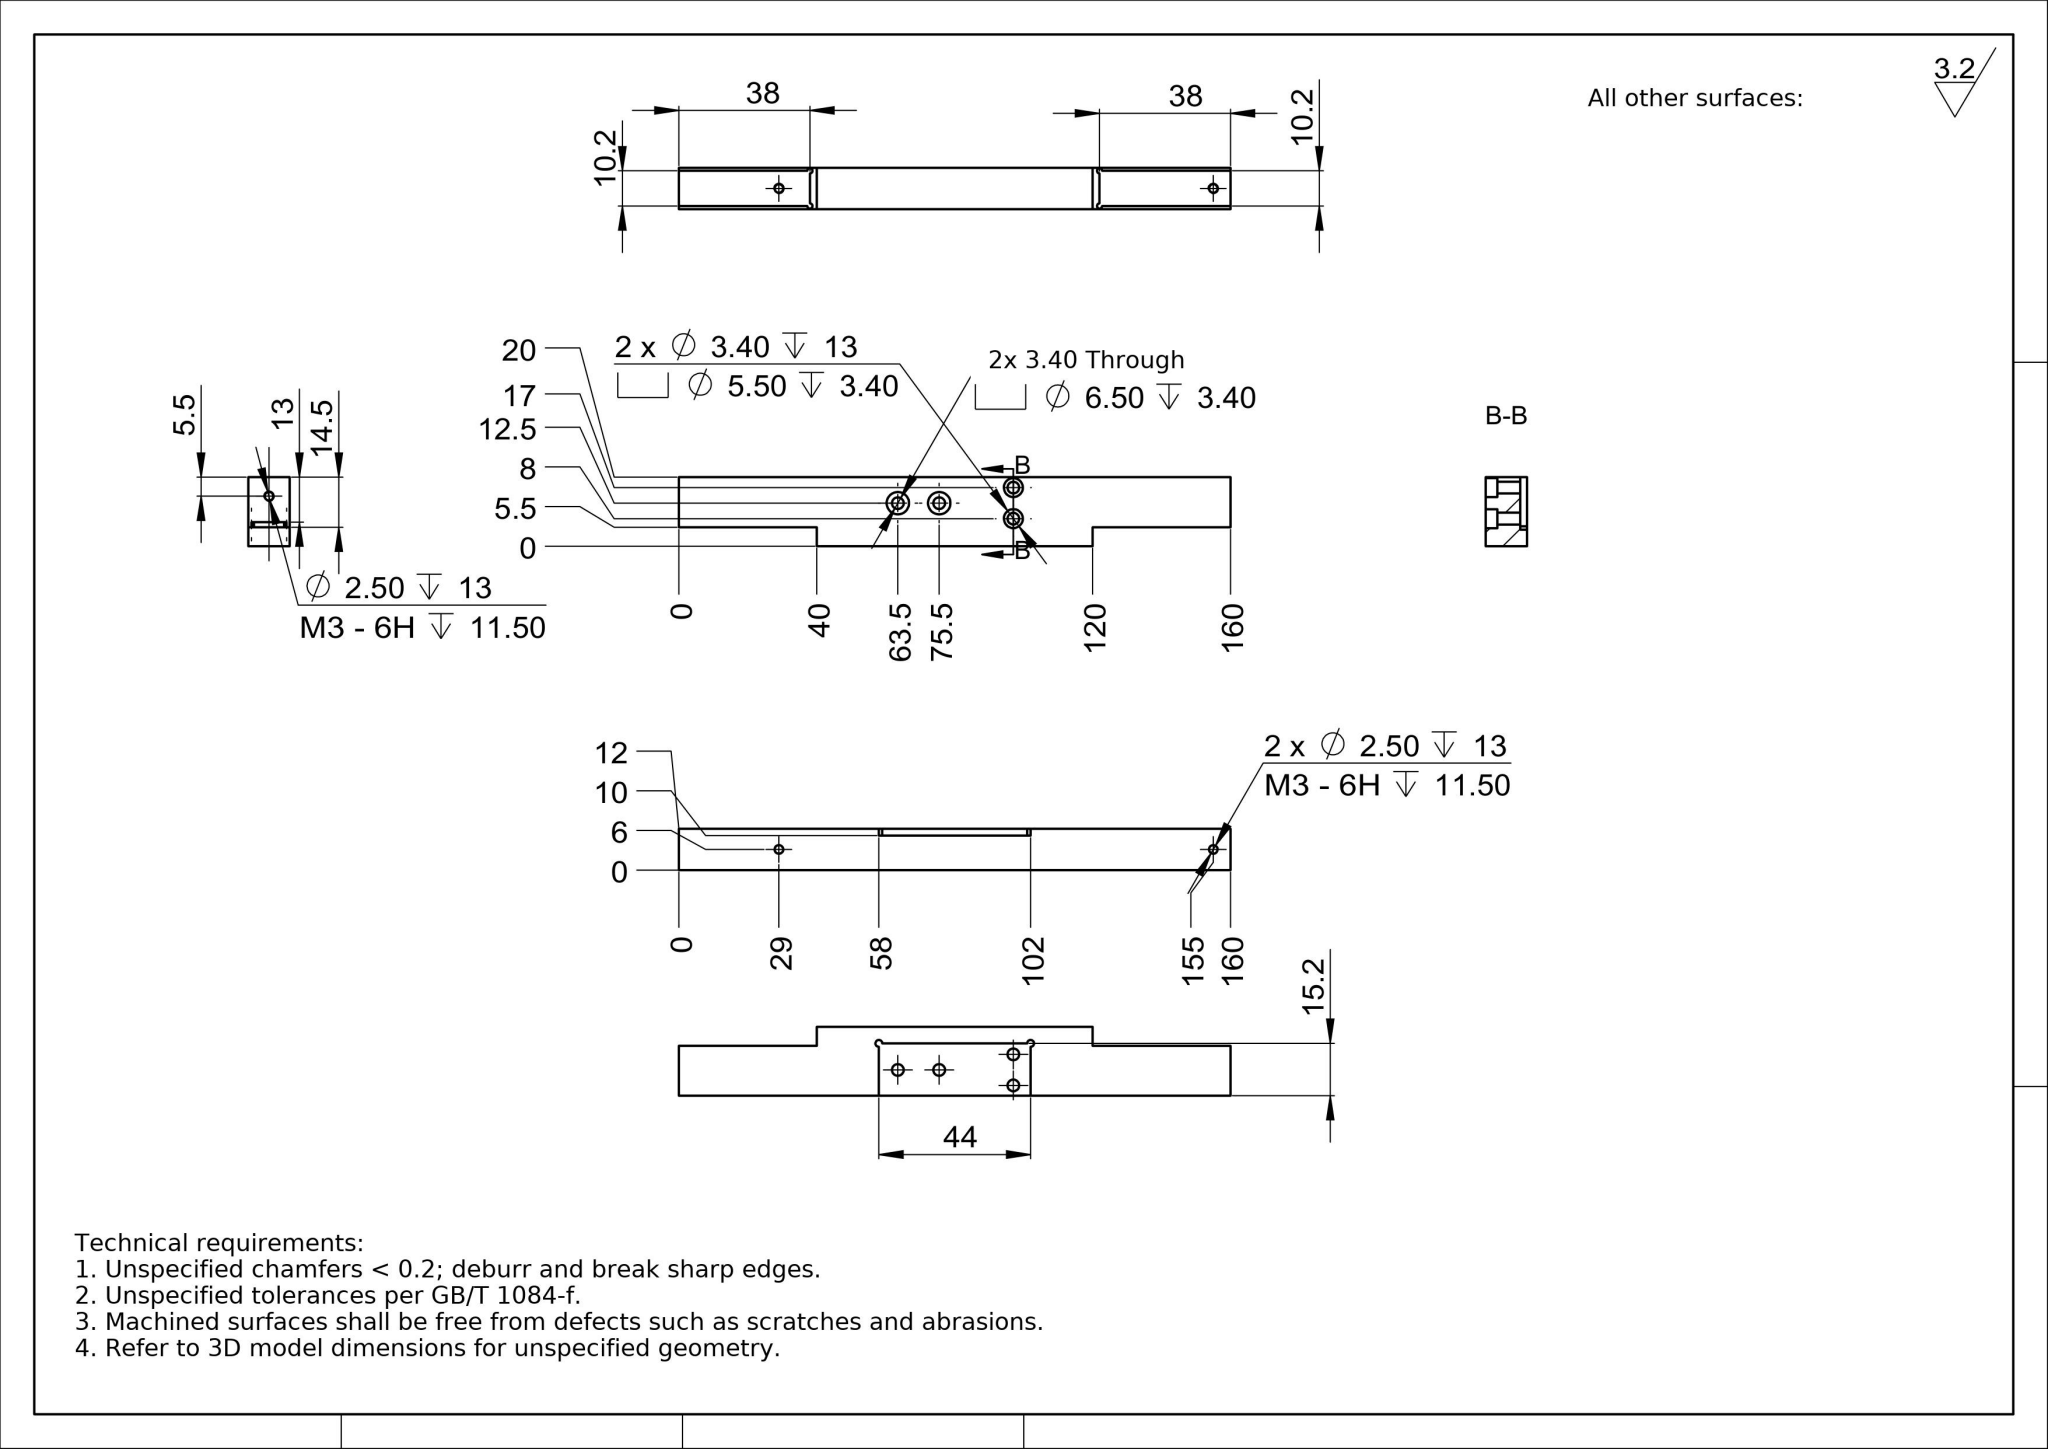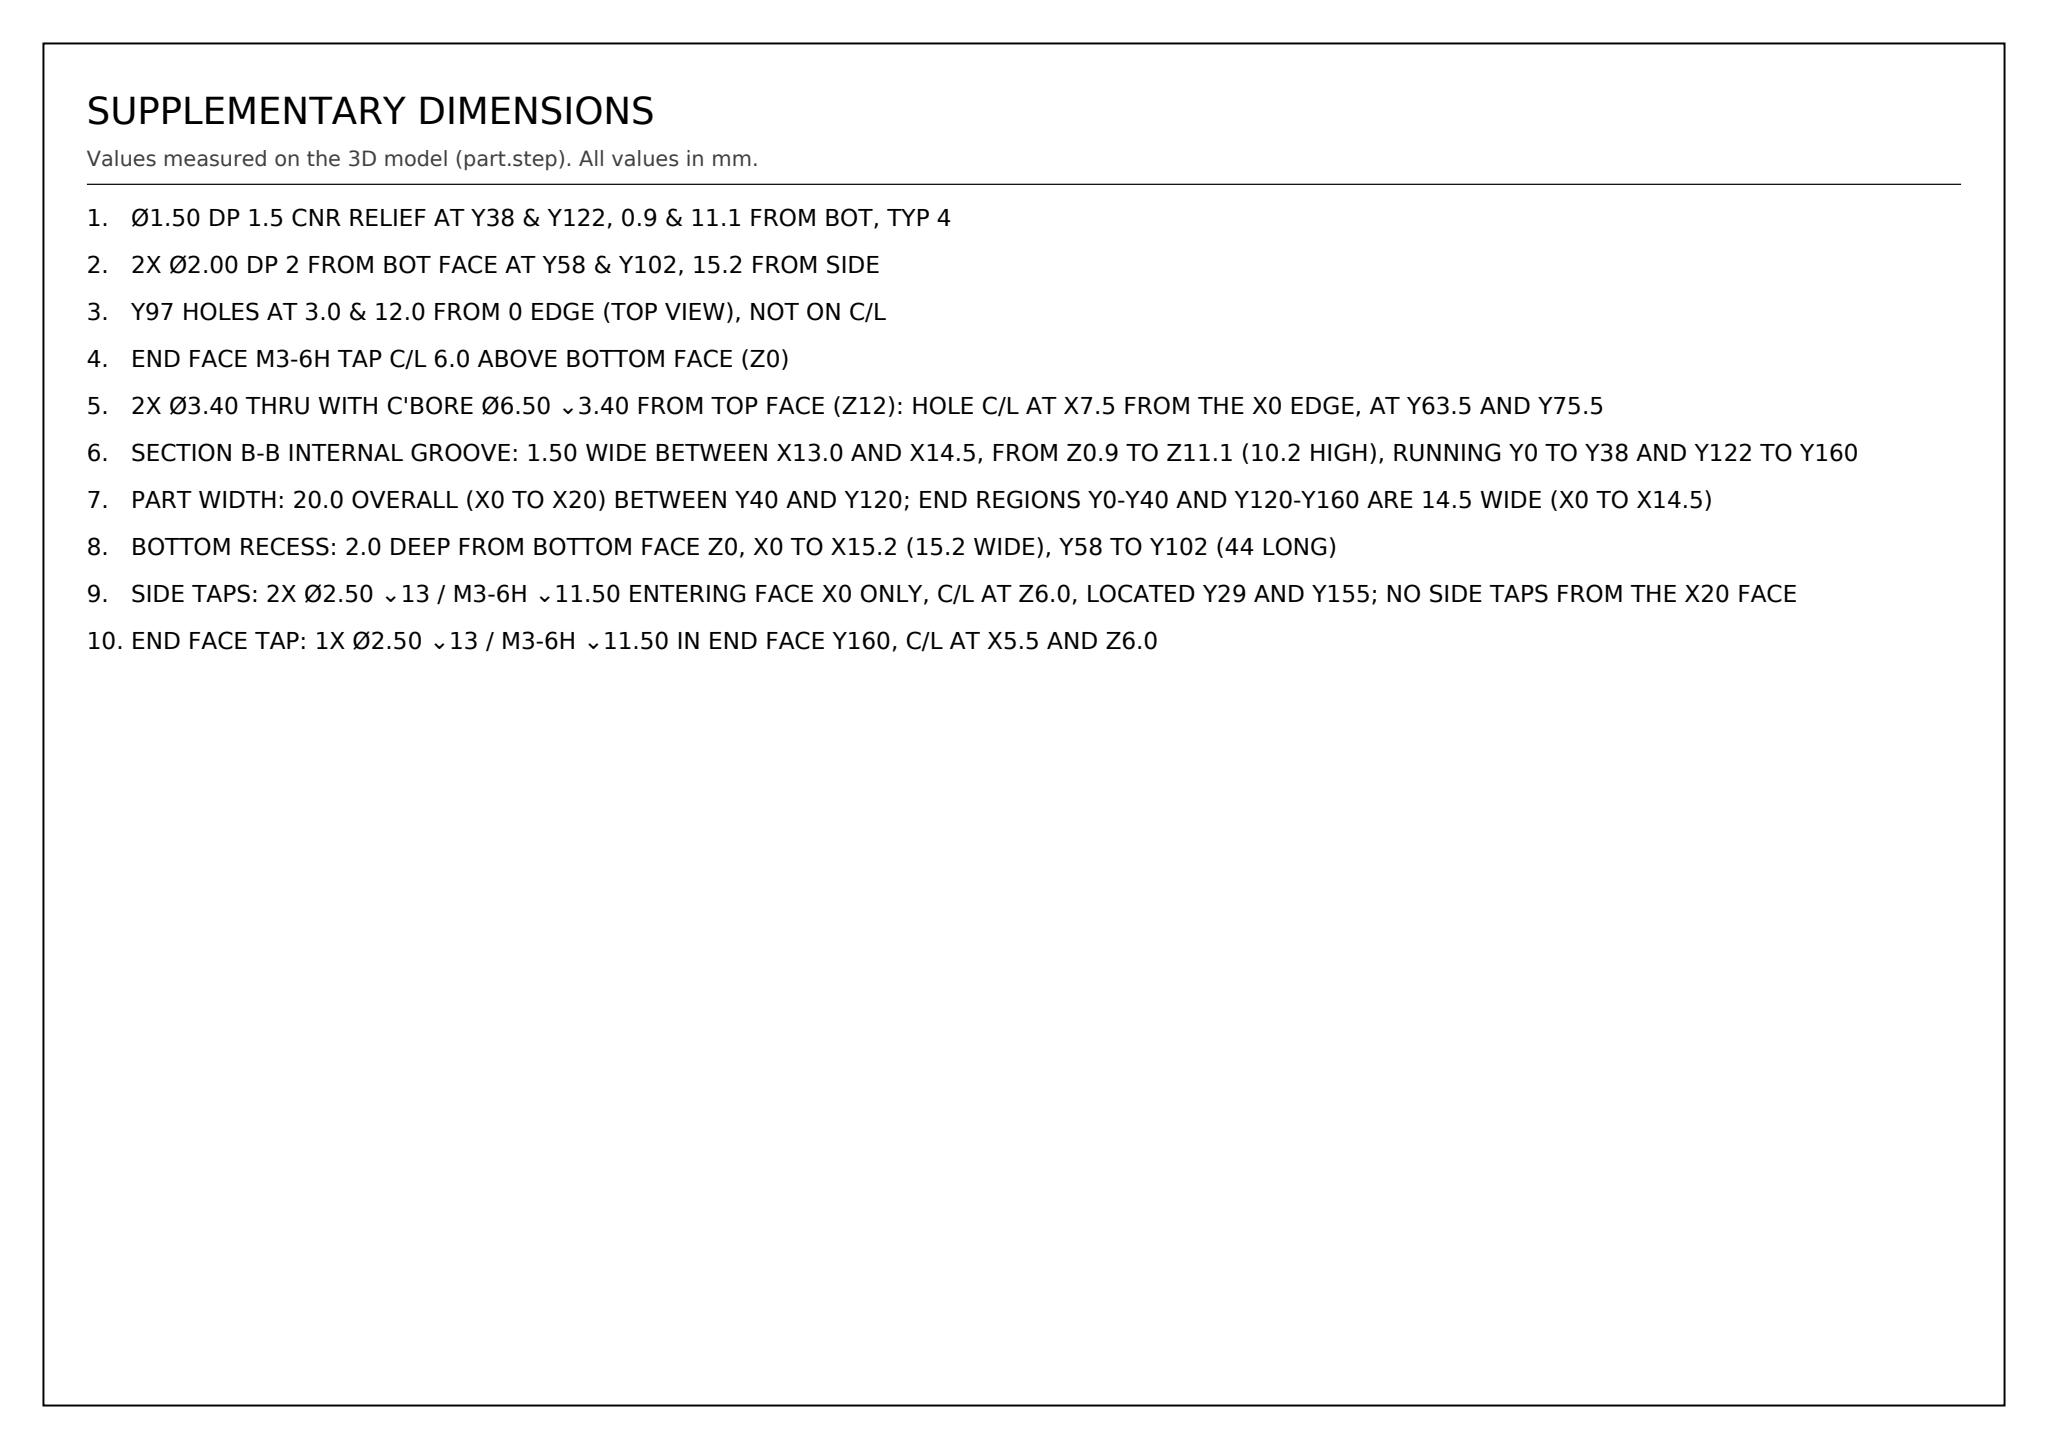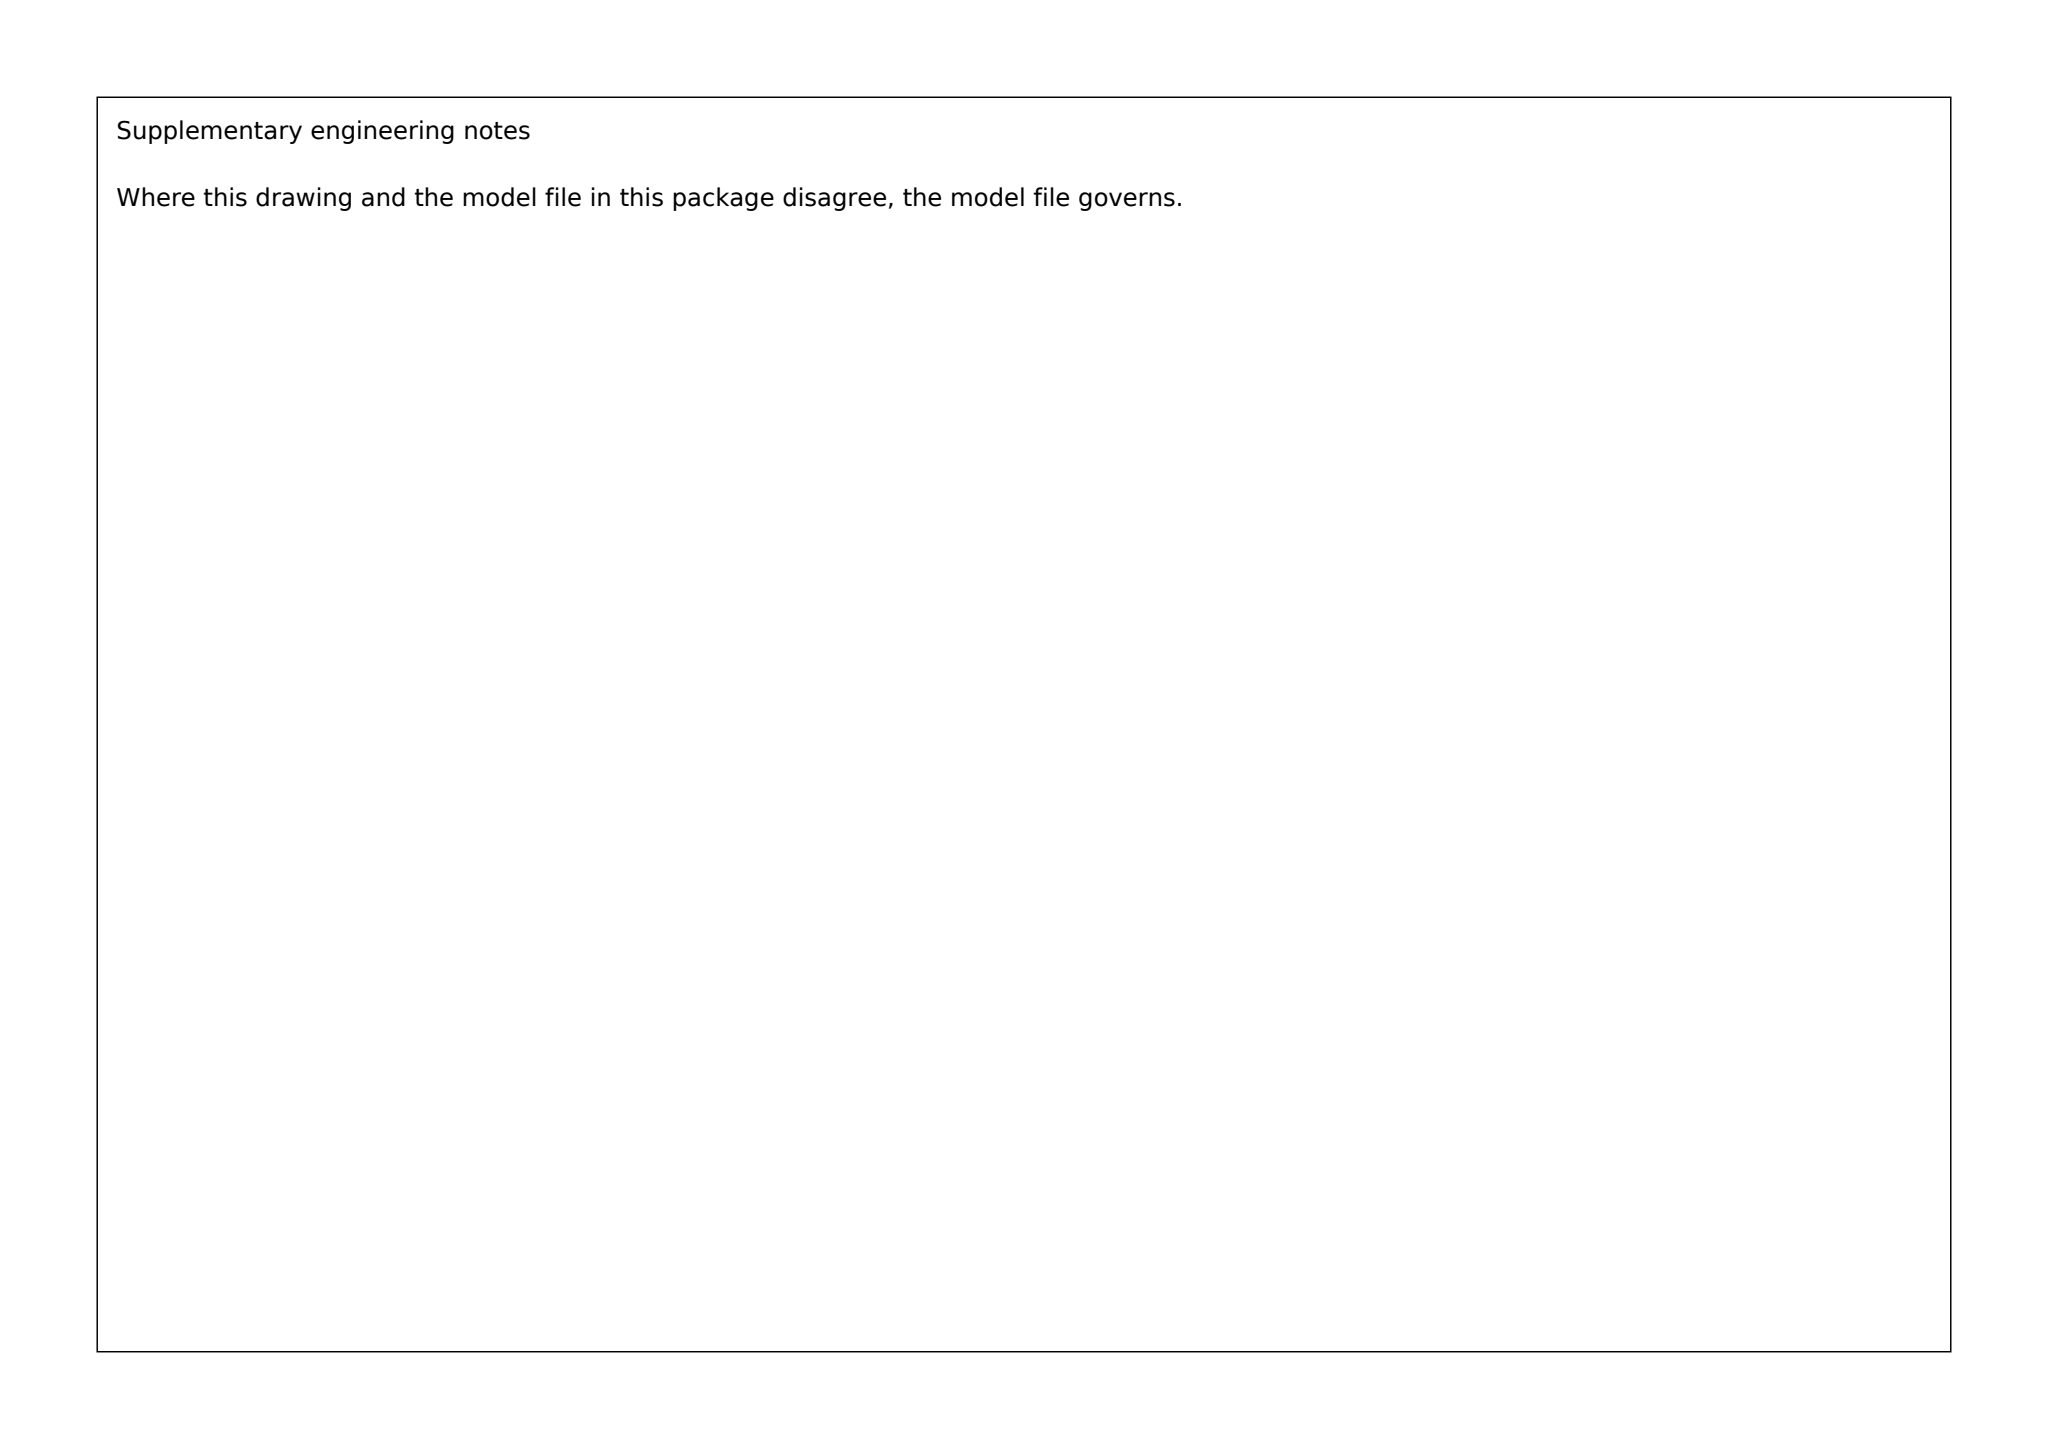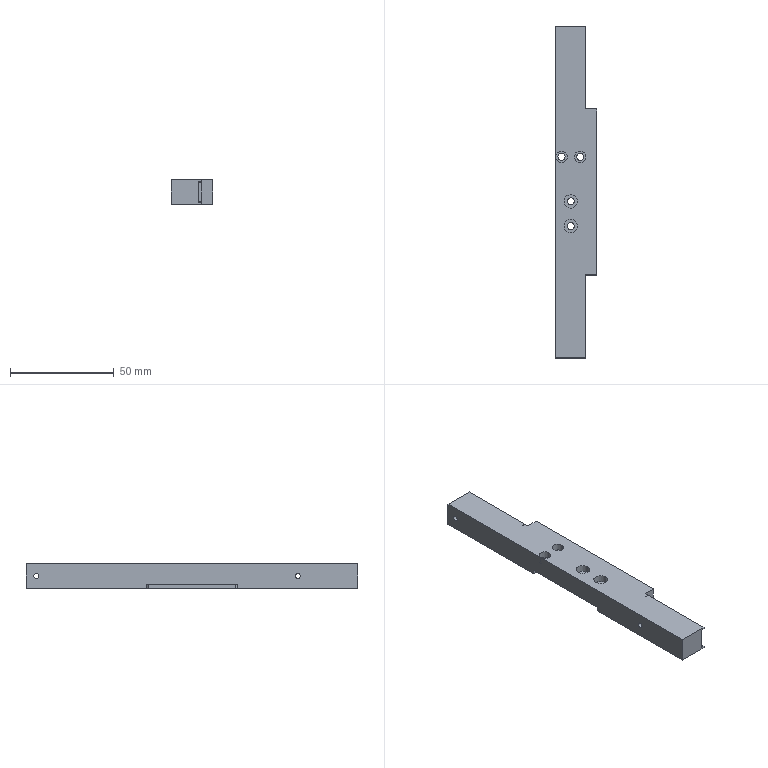Part | SolidWorks | mm | 1 solid | 62 faces | box 20 x 160 x 12 mm | volume 29793 mm3 | cylinder 34 | plane 26 | cone 2 | commonest cylinder face diameters 2.5 x10 3.4 x8 1.5 x6 6.5 x4 5.5 x4 2 x2
Drawing notes:
Ø1.50 DP 1.5 CNR RELIEF AT Y38 & Y122, 0.9 & 11.1 FROM BOT, TYP 4 | from the solid: Ø1.5 x-axis cyls len 1.5 at y=38 & 122, z=0.9 & 11.1
2X Ø2.00 DP 2 FROM BOT FACE AT Y58 & Y102, 15.2 FROM SIDE | from the solid: Ø2.0 z cyls at [15.2,58] & [15.2,102], len 2.0; plane z=2.0
Y97 HOLES AT 3.0 & 12.0 FROM 0 EDGE (TOP VIEW), NOT ON C/L | from the solid: Ø3.4/Ø5.5 z-holes at x=3.0 and x=12.0, y=97.0
END FACE M3-6H TAP C/L 6.0 ABOVE BOTTOM FACE (Z0) | from the solid: Ø2.5 y-axis hole at z=6.0, x=5.5
2X Ø3.40 THRU WITH C'BORE Ø6.50 ⌄3.40 FROM TOP FACE (Z12): HOLE C/L AT X7.5 FROM THE X0 EDGE, AT Y63.5 AND Y75.5 | from the solid: cylinders: Ø3.4 axis z at [7.5, 63.5] and [7.5, 75.5] from Z2.0 to 8.6; Ø6.5 same axes from Z8.6 to 12.0
SECTION B-B INTERNAL GROOVE: 1.50 WIDE BETWEEN X13.0 AND X14.5, FROM Z0.9 TO Z11.1 (10.2 HIGH), RUNNING Y0 TO Y38 AND Y122 TO Y160 | from the solid: axis_planes x=13.0 (y0-38.8 and y121.2-160, z0.1-11.9), x=14.5, and z=0.9 / z=11.1 each x13.0-14.5
PART WIDTH: 20.0 OVERALL (X0 TO X20) BETWEEN Y40 AND Y120; END REGIONS Y0-Y40 AND Y120-Y160 ARE 14.5 WIDE (X0 TO X14.5) | from the solid: axis_planes x=20.0 extent y40-120 z0-12; x=14.5 extents y0-40 and y120-160, z0-12
BOTTOM RECESS: 2.0 DEEP FROM BOTTOM FACE Z0, X0 TO X15.2 (15.2 WIDE), Y58 TO Y102 (44 LONG) | from the solid: axis_plane z=2.0 (x0-16.2, y57-103); x=15.2 (y59-101, z0-2); y=58 and y=102 (x0-14.2, z0-2)
SIDE TAPS: 2X Ø2.50 ⌄13 / M3-6H ⌄11.50 ENTERING FACE X0 ONLY, C/L AT Z6.0, LOCATED Y29 AND Y155; NO SIDE TAPS FROM THE X20 FACE | from the solid: cylinders Ø2.5 axis x at [y155, z6.0] from x0-5.5 and x5.5-13.0, and at [y29, z6.0] from x0-13.0
END FACE TAP: 1X Ø2.50 ⌄13 / M3-6H ⌄11.50 IN END FACE Y160, C/L AT X5.5 AND Z6.0 | from the solid: cylinders Ø2.5 axis y at [x5.5, z6.0] from y155-160 and y147-155; cones 118° ref Ø2.5 at y146.2
build123d program:
from build123d import *

# Parameters (mm, degrees)
SKETCH1_W                                       = 20
SKETCH1_H                                       = 160
BOSS_EXTRUDE1_DEPTH                             = 6
SKETCH3_W                                       = 12
SKETCH3_H                                       = 40
CUT_EXTRUDE2_DEPTH                              = 5.5
SKETCH4_W                                       = 15.2
SKETCH4_H                                       = 44
CUT_EXTRUDE3_DEPTH                              = 2
SKETCH5_W                                       = 10.2
SKETCH5_H                                       = 38
CUT_EXTRUDE4_DEPTH                              = 1.5
M3_TAPPED_HOLE1_D                               = 2.5
M3_TAPPED_HOLE1_DEPTH                           = 13
M3_TAPPED_HOLE1_TIP                             = 0.7511
M3_TAPPED_HOLE2_D                               = 2.5
M3_TAPPED_HOLE2_DEPTH                           = 13
M3_TAPPED_HOLE2_TIP                             = 0.7511
M3_HEX_SOCKET_HEAD_CAP_SCREW_CBORE3_D           = 3.4
M3_HEX_SOCKET_HEAD_CAP_SCREW_CBORE3_DEPTH       = 13
M3_HEX_SOCKET_HEAD_CAP_SCREW_CBORE3_CBORE_D     = 5.5
M3_HEX_SOCKET_HEAD_CAP_SCREW_CBORE3_CBORE_DEPTH = 3.4
M3_HEX_SOCKET_HEAD_CAP_SCREW_CBORE3_TIP         = 1.021
M3_HEX_SOCKET_HEAD_CAP_SCREW_CBORE4_D           = 3.4
M3_HEX_SOCKET_HEAD_CAP_SCREW_CBORE4_CBORE_D     = 6.5
M3_HEX_SOCKET_HEAD_CAP_SCREW_CBORE4_CBORE_DEPTH = 3.4
F_1_5_1_5_DIAMETER_HOLE1_AT_2_COUNT             = 2
F_1_5_1_5_DIAMETER_HOLE1_AT_2_PITCH             = 10.2
F_1_5_1_5_DIAMETER_HOLE1_AT_3_COUNT             = 2
F_1_5_1_5_DIAMETER_HOLE1_AT_3_PITCH             = 84
F_1_5_1_5_DIAMETER_HOLE1_AT_4_COUNT             = 2
F_1_5_1_5_DIAMETER_HOLE1_AT_4_PITCH             = 84.617
SKETCH18_R                                      = 1
CUT_EXTRUDE5_DEPTH                              = 2


with BuildPart() as part:
    # Sketch1 → Boss-Extrude1 (new, symmetric)
    with BuildSketch(Plane.XY):
        Rectangle(SKETCH1_W, SKETCH1_H)
    extrude(amount=BOSS_EXTRUDE1_DEPTH, both=True)

    # Sketch3 → Cut-Extrude2 (cut)
    with BuildSketch(Plane(origin=(10, 0, 0), x_dir=(0, 0, -1), z_dir=(1, 0, 0))):
        with Locations((0, -60)):
            Rectangle(SKETCH3_W, SKETCH3_H)
        with Locations((0, 60)):
            Rectangle(SKETCH3_W, SKETCH3_H)
    extrude(amount=-CUT_EXTRUDE2_DEPTH, mode=Mode.SUBTRACT)

    # Sketch4 → Cut-Extrude3 (cut)
    with BuildSketch(Plane(origin=(0, 0, -6), x_dir=(-1, 0, 0), z_dir=(0, 0, -1))):
        with Locations((2.4, 0)):
            Rectangle(SKETCH4_W, SKETCH4_H)
    extrude(amount=-CUT_EXTRUDE3_DEPTH, mode=Mode.SUBTRACT)

    # Sketch5 → Cut-Extrude4 (cut)
    with BuildSketch(Plane(origin=(4.5, 0, 0), x_dir=(0, 0, -1), z_dir=(1, 0, 0))):
        with Locations((0, -61)):
            Rectangle(SKETCH5_W, SKETCH5_H)
        with Locations((0, 61)):
            Rectangle(SKETCH5_W, SKETCH5_H)
    extrude(amount=-CUT_EXTRUDE4_DEPTH, mode=Mode.SUBTRACT)

    # M3 Tapped Hole1
    with Locations(Plane(origin=(0, 80, 0), x_dir=(1, 0, 0), z_dir=(0, 1, 0))):
        with Locations((-4.5, 0)):
            Hole(M3_TAPPED_HOLE1_D / 2, depth=M3_TAPPED_HOLE1_DEPTH)
            with Locations((0, 0, -(M3_TAPPED_HOLE1_DEPTH + M3_TAPPED_HOLE1_TIP / 2))):  # 118° drill point
                Cone(0, M3_TAPPED_HOLE1_D / 2, M3_TAPPED_HOLE1_TIP, mode=Mode.SUBTRACT)

    # M3 Tapped Hole2
    with Locations(Plane(origin=(3, 0, 0), x_dir=(0, 0, -1), z_dir=(1, 0, 0))):
        with Locations((0, 75), (0, -51)):
            Hole(M3_TAPPED_HOLE2_D / 2, depth=M3_TAPPED_HOLE2_DEPTH)
            with Locations((0, 0, -(M3_TAPPED_HOLE2_DEPTH + M3_TAPPED_HOLE2_TIP / 2))):  # 118° drill point
                Cone(0, M3_TAPPED_HOLE2_D / 2, M3_TAPPED_HOLE2_TIP, mode=Mode.SUBTRACT)

    # M3 Hex Socket Head Cap Screw CBORE3
    with Locations(Plane.XY.offset(6)):
        with Locations((-7, 17), (2, 17)):
            CounterBoreHole(M3_HEX_SOCKET_HEAD_CAP_SCREW_CBORE3_D / 2, M3_HEX_SOCKET_HEAD_CAP_SCREW_CBORE3_CBORE_D / 2, M3_HEX_SOCKET_HEAD_CAP_SCREW_CBORE3_CBORE_DEPTH, depth=M3_HEX_SOCKET_HEAD_CAP_SCREW_CBORE3_DEPTH)
            with Locations((0, 0, -(M3_HEX_SOCKET_HEAD_CAP_SCREW_CBORE3_DEPTH + M3_HEX_SOCKET_HEAD_CAP_SCREW_CBORE3_TIP / 2))):  # 118° drill point
                Cone(0, M3_HEX_SOCKET_HEAD_CAP_SCREW_CBORE3_D / 2, M3_HEX_SOCKET_HEAD_CAP_SCREW_CBORE3_TIP, mode=Mode.SUBTRACT)

    # M3 Hex Socket Head Cap Screw CBORE4 (through all)
    with Locations(Plane.XY.offset(6)):
        with Locations((-2.5, -4.5), (-2.5, -16.5)):
            CounterBoreHole(M3_HEX_SOCKET_HEAD_CAP_SCREW_CBORE4_D / 2, M3_HEX_SOCKET_HEAD_CAP_SCREW_CBORE4_CBORE_D / 2, M3_HEX_SOCKET_HEAD_CAP_SCREW_CBORE4_CBORE_DEPTH)

    # Sketch17 → 1.5 _1.5_ Diameter Hole1 (revolve, cut)
    with BuildSketch(Plane(origin=(3, 42, 5.1), x_dir=(0, 0, 1), z_dir=(0, 1, 0))):
        Polygon((0, 0), (0, 10.551), (0.75, 10.1), (0.75, 0), align=None)
    f_1_5_1_5_diameter_hole1 = revolve(axis=Axis((-3.35, 42, 5.1), (1, 0, 0)), mode=Mode.SUBTRACT)

    # 1.5 _1.5_ Diameter Hole1 at 2: 1.5 _1.5_ Diameter Hole1 ×2
    with Locations(*[(0, 0, -i * F_1_5_1_5_DIAMETER_HOLE1_AT_2_PITCH) for i in range(1, F_1_5_1_5_DIAMETER_HOLE1_AT_2_COUNT)]):
        add(f_1_5_1_5_diameter_hole1, mode=Mode.SUBTRACT)

    # 1.5 _1.5_ Diameter Hole1 at 3: 1.5 _1.5_ Diameter Hole1 ×2
    with Locations(*[(0, -i * F_1_5_1_5_DIAMETER_HOLE1_AT_3_PITCH, 0) for i in range(1, F_1_5_1_5_DIAMETER_HOLE1_AT_3_COUNT)]):
        add(f_1_5_1_5_diameter_hole1, mode=Mode.SUBTRACT)

    # 1.5 _1.5_ Diameter Hole1 at 4: 1.5 _1.5_ Diameter Hole1 ×2
    with Locations(*[Vector(0, -0.9927, -0.1205) * (i * F_1_5_1_5_DIAMETER_HOLE1_AT_4_PITCH) for i in range(1, F_1_5_1_5_DIAMETER_HOLE1_AT_4_COUNT)]):
        add(f_1_5_1_5_diameter_hole1, mode=Mode.SUBTRACT)

    # Sketch18 → Cut-Extrude5 (cut)
    with BuildSketch(Plane(origin=(0, 0, -6), x_dir=(-1, 0, 0), z_dir=(0, 0, -1))):
        with Locations((-5.2, 22)):
            Circle(SKETCH18_R)
        with Locations((-5.2, -22)):
            Circle(SKETCH18_R)
    extrude(amount=-CUT_EXTRUDE5_DEPTH, mode=Mode.SUBTRACT)


solid = part.part